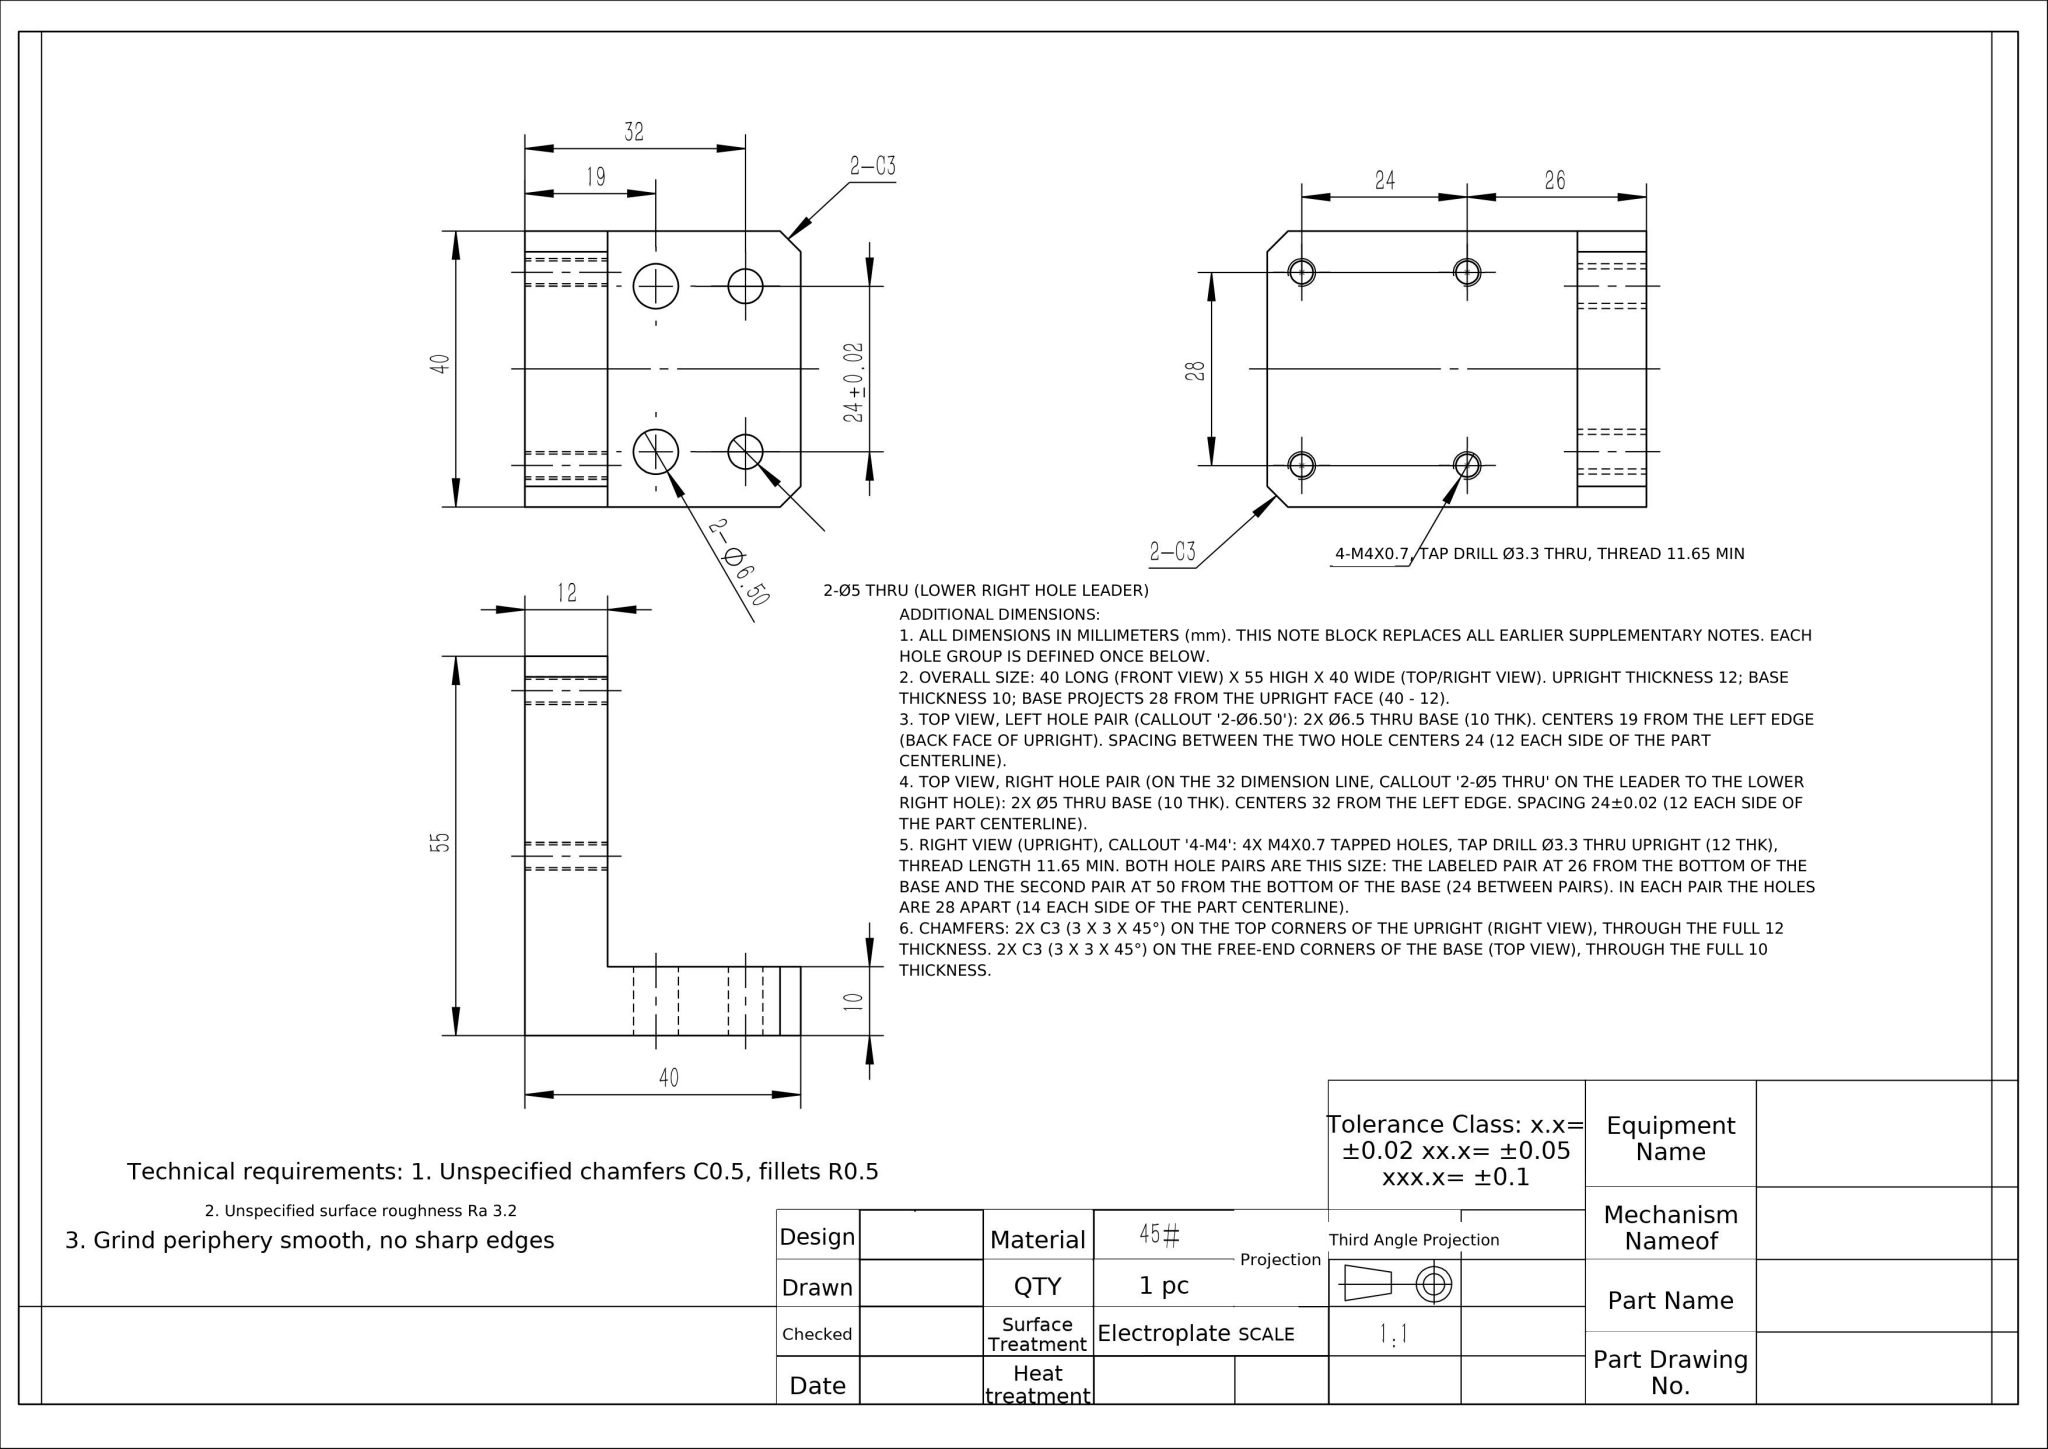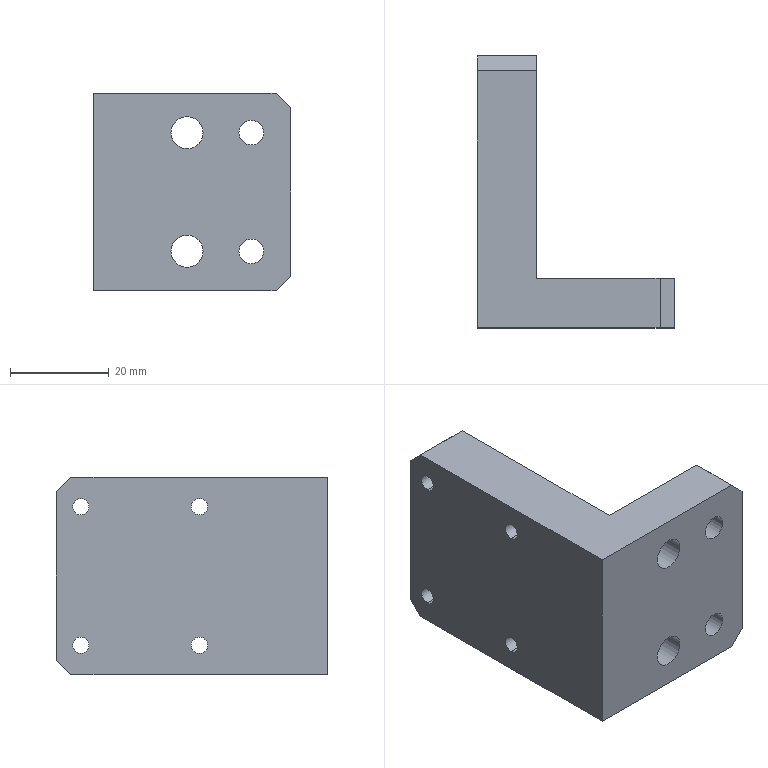Part | NX | mm | 1 solid | 28 faces | box 40 x 55 x 40 mm | volume 35935 mm3 | cylinder 16 | plane 12 | commonest cylinder face diameters 3.3 x8 6.5 x4 5 x4
STEP:
#1=CARTESIAN_POINT('',(12.,50.,-15.65));
#2=VERTEX_POINT('',#1);
#3=CARTESIAN_POINT('',(12.,50.,-12.35));
#4=VERTEX_POINT('',#3);
#5=CARTESIAN_POINT('',(12.,50.,-14.));
#6=DIRECTION('',(-1.,0.,0.));
#7=DIRECTION('',(0.,0.,1.));
#8=AXIS2_PLACEMENT_3D('',#5,#6,#7);
#9=CIRCLE('',#8,1.65);
#10=EDGE_CURVE('',#2,#4,#9,.T.);
#11=ORIENTED_EDGE('',*,*,#10,.F.);
#12=CARTESIAN_POINT('',(-0.,50.,-15.65));
#13=VERTEX_POINT('',#12);
#14=CARTESIAN_POINT('',(0.,50.,-15.65));
#15=DIRECTION('',(-1.,0.,0.));
#16=VECTOR('',#15,1000.);
#17=LINE('',#14,#16);
#18=EDGE_CURVE('',#2,#13,#17,.T.);
#19=ORIENTED_EDGE('',*,*,#18,.T.);
#20=CARTESIAN_POINT('',(-0.,50.,-12.35));
#21=VERTEX_POINT('',#20);
#22=CARTESIAN_POINT('',(-0.,50.,-14.));
#23=DIRECTION('',(-1.,0.,0.));
#24=DIRECTION('',(0.,0.,1.));
#25=AXIS2_PLACEMENT_3D('',#22,#23,#24);
#26=CIRCLE('',#25,1.65);
#27=EDGE_CURVE('',#13,#21,#26,.T.);
#28=ORIENTED_EDGE('',*,*,#27,.T.);
#29=CARTESIAN_POINT('',(0.,50.,-12.35));
#30=DIRECTION('',(-1.,0.,0.));
#31=VECTOR('',#30,1000.);
#32=LINE('',#29,#31);
#33=EDGE_CURVE('',#4,#21,#32,.T.);
#34=ORIENTED_EDGE('',*,*,#33,.F.);
#35=EDGE_LOOP('',(#11,#19,#28,#34));
#36=FACE_OUTER_BOUND('',#35,.T.);
#37=CARTESIAN_POINT('',(0.,50.,-14.));
#38=DIRECTION('',(-1.,0.,0.));
#39=DIRECTION('',(0.,0.,1.));
#40=AXIS2_PLACEMENT_3D('',#37,#38,#39);
#41=CYLINDRICAL_SURFACE('',#40,1.65);
#42=ADVANCED_FACE('',(#36),#41,.F.);
#43=CARTESIAN_POINT('',(12.,50.,12.35));
#44=VERTEX_POINT('',#43);
#45=CARTESIAN_POINT('',(12.,50.,15.65));
#46=VERTEX_POINT('',#45);
#47=CARTESIAN_POINT('',(12.,50.,14.));
#48=DIRECTION('',(-1.,0.,0.));
#49=DIRECTION('',(0.,0.,1.));
#50=AXIS2_PLACEMENT_3D('',#47,#48,#49);
#51=CIRCLE('',#50,1.65);
#52=EDGE_CURVE('',#44,#46,#51,.T.);
#53=ORIENTED_EDGE('',*,*,#52,.F.);
#54=CARTESIAN_POINT('',(-0.,50.,12.35));
#55=VERTEX_POINT('',#54);
#56=CARTESIAN_POINT('',(0.,50.,12.35));
#57=DIRECTION('',(-1.,0.,0.));
#58=VECTOR('',#57,1000.);
#59=LINE('',#56,#58);
#60=EDGE_CURVE('',#44,#55,#59,.T.);
#61=ORIENTED_EDGE('',*,*,#60,.T.);
#62=CARTESIAN_POINT('',(-0.,50.,15.65));
#63=VERTEX_POINT('',#62);
#64=CARTESIAN_POINT('',(-0.,50.,14.));
#65=DIRECTION('',(-1.,0.,0.));
#66=DIRECTION('',(0.,0.,1.));
#67=AXIS2_PLACEMENT_3D('',#64,#65,#66);
#68=CIRCLE('',#67,1.65);
#69=EDGE_CURVE('',#55,#63,#68,.T.);
#70=ORIENTED_EDGE('',*,*,#69,.T.);
#71=CARTESIAN_POINT('',(0.,50.,15.65));
#72=DIRECTION('',(-1.,0.,0.));
#73=VECTOR('',#72,1000.);
#74=LINE('',#71,#73);
#75=EDGE_CURVE('',#46,#63,#74,.T.);
#76=ORIENTED_EDGE('',*,*,#75,.F.);
#77=EDGE_LOOP('',(#53,#61,#70,#76));
#78=FACE_OUTER_BOUND('',#77,.T.);
#79=CARTESIAN_POINT('',(0.,50.,14.));
#80=DIRECTION('',(-1.,0.,0.));
#81=DIRECTION('',(0.,0.,1.));
#82=AXIS2_PLACEMENT_3D('',#79,#80,#81);
#83=CYLINDRICAL_SURFACE('',#82,1.65);
#84=ADVANCED_FACE('',(#78),#83,.F.);
#85=CARTESIAN_POINT('',(12.,26.,12.35));
#86=VERTEX_POINT('',#85);
#87=CARTESIAN_POINT('',(12.,26.,15.65));
#88=VERTEX_POINT('',#87);
#89=CARTESIAN_POINT('',(12.,26.,14.));
#90=DIRECTION('',(-1.,0.,0.));
#91=DIRECTION('',(0.,0.,1.));
#92=AXIS2_PLACEMENT_3D('',#89,#90,#91);
#93=CIRCLE('',#92,1.65);
#94=EDGE_CURVE('',#86,#88,#93,.T.);
#95=ORIENTED_EDGE('',*,*,#94,.F.);
#96=CARTESIAN_POINT('',(-0.,26.,12.35));
#97=VERTEX_POINT('',#96);
#98=CARTESIAN_POINT('',(0.,26.,12.35));
#99=DIRECTION('',(-1.,0.,0.));
#100=VECTOR('',#99,1000.);
#101=LINE('',#98,#100);
#102=EDGE_CURVE('',#86,#97,#101,.T.);
#103=ORIENTED_EDGE('',*,*,#102,.T.);
#104=CARTESIAN_POINT('',(-0.,26.,15.65));
#105=VERTEX_POINT('',#104);
#106=CARTESIAN_POINT('',(-0.,26.,14.));
#107=DIRECTION('',(-1.,0.,0.));
#108=DIRECTION('',(0.,0.,1.));
#109=AXIS2_PLACEMENT_3D('',#106,#107,#108);
#110=CIRCLE('',#109,1.65);
#111=EDGE_CURVE('',#97,#105,#110,.T.);
#112=ORIENTED_EDGE('',*,*,#111,.T.);
#113=CARTESIAN_POINT('',(0.,26.,15.65));
#114=DIRECTION('',(-1.,0.,0.));
#115=VECTOR('',#114,1000.);
#116=LINE('',#113,#115);
#117=EDGE_CURVE('',#88,#105,#116,.T.);
#118=ORIENTED_EDGE('',*,*,#117,.F.);
#119=EDGE_LOOP('',(#95,#103,#112,#118));
#120=FACE_OUTER_BOUND('',#119,.T.);
#121=CARTESIAN_POINT('',(0.,26.,14.));
#122=DIRECTION('',(-1.,0.,0.));
#123=DIRECTION('',(0.,0.,1.));
#124=AXIS2_PLACEMENT_3D('',#121,#122,#123);
#125=CYLINDRICAL_SURFACE('',#124,1.65);
#126=ADVANCED_FACE('',(#120),#125,.F.);
#127=CARTESIAN_POINT('',(12.,26.,-15.65));
#128=VERTEX_POINT('',#127);
#129=CARTESIAN_POINT('',(12.,26.,-12.35));
#130=VERTEX_POINT('',#129);
#131=CARTESIAN_POINT('',(12.,26.,-14.));
#132=DIRECTION('',(-1.,0.,0.));
#133=DIRECTION('',(0.,0.,1.));
#134=AXIS2_PLACEMENT_3D('',#131,#132,#133);
#135=CIRCLE('',#134,1.65);
#136=EDGE_CURVE('',#128,#130,#135,.T.);
#137=ORIENTED_EDGE('',*,*,#136,.F.);
#138=CARTESIAN_POINT('',(-0.,26.,-15.65));
#139=VERTEX_POINT('',#138);
#140=CARTESIAN_POINT('',(0.,26.,-15.65));
#141=DIRECTION('',(-1.,0.,0.));
#142=VECTOR('',#141,1000.);
#143=LINE('',#140,#142);
#144=EDGE_CURVE('',#128,#139,#143,.T.);
#145=ORIENTED_EDGE('',*,*,#144,.T.);
#146=CARTESIAN_POINT('',(-0.,26.,-12.35));
#147=VERTEX_POINT('',#146);
#148=CARTESIAN_POINT('',(-0.,26.,-14.));
#149=DIRECTION('',(-1.,0.,0.));
#150=DIRECTION('',(0.,0.,1.));
#151=AXIS2_PLACEMENT_3D('',#148,#149,#150);
#152=CIRCLE('',#151,1.65);
#153=EDGE_CURVE('',#139,#147,#152,.T.);
#154=ORIENTED_EDGE('',*,*,#153,.T.);
#155=CARTESIAN_POINT('',(0.,26.,-12.35));
#156=DIRECTION('',(-1.,0.,0.));
#157=VECTOR('',#156,1000.);
#158=LINE('',#155,#157);
#159=EDGE_CURVE('',#130,#147,#158,.T.);
#160=ORIENTED_EDGE('',*,*,#159,.F.);
#161=EDGE_LOOP('',(#137,#145,#154,#160));
#162=FACE_OUTER_BOUND('',#161,.T.);
#163=CARTESIAN_POINT('',(0.,26.,-14.));
#164=DIRECTION('',(-1.,0.,0.));
#165=DIRECTION('',(0.,0.,1.));
#166=AXIS2_PLACEMENT_3D('',#163,#164,#165);
#167=CYLINDRICAL_SURFACE('',#166,1.65);
#168=ADVANCED_FACE('',(#162),#167,.F.);
#169=CARTESIAN_POINT('',(22.25,-0.,12.));
#170=VERTEX_POINT('',#169);
#171=CARTESIAN_POINT('',(15.75,-0.,12.));
#172=VERTEX_POINT('',#171);
#173=CARTESIAN_POINT('',(19.,-0.,12.));
#174=DIRECTION('',(-0.,1.,0.));
#175=DIRECTION('',(1.,0.,0.));
#176=AXIS2_PLACEMENT_3D('',#173,#174,#175);
#177=CIRCLE('',#176,3.25);
#178=EDGE_CURVE('',#170,#172,#177,.T.);
#179=ORIENTED_EDGE('',*,*,#178,.F.);
#180=CARTESIAN_POINT('',(22.25,10.,12.));
#181=VERTEX_POINT('',#180);
#182=CARTESIAN_POINT('',(22.25,-0.,12.));
#183=DIRECTION('',(-0.,1.,0.));
#184=VECTOR('',#183,1000.);
#185=LINE('',#182,#184);
#186=EDGE_CURVE('',#170,#181,#185,.T.);
#187=ORIENTED_EDGE('',*,*,#186,.T.);
#188=CARTESIAN_POINT('',(15.75,10.,12.));
#189=VERTEX_POINT('',#188);
#190=CARTESIAN_POINT('',(19.,10.,12.));
#191=DIRECTION('',(-0.,1.,0.));
#192=DIRECTION('',(1.,0.,0.));
#193=AXIS2_PLACEMENT_3D('',#190,#191,#192);
#194=CIRCLE('',#193,3.25);
#195=EDGE_CURVE('',#181,#189,#194,.T.);
#196=ORIENTED_EDGE('',*,*,#195,.T.);
#197=CARTESIAN_POINT('',(15.75,-0.,12.));
#198=DIRECTION('',(-0.,1.,0.));
#199=VECTOR('',#198,1000.);
#200=LINE('',#197,#199);
#201=EDGE_CURVE('',#172,#189,#200,.T.);
#202=ORIENTED_EDGE('',*,*,#201,.F.);
#203=EDGE_LOOP('',(#179,#187,#196,#202));
#204=FACE_OUTER_BOUND('',#203,.T.);
#205=CARTESIAN_POINT('',(19.,-0.,12.));
#206=DIRECTION('',(-0.,1.,0.));
#207=DIRECTION('',(-1.,-0.,0.));
#208=AXIS2_PLACEMENT_3D('',#205,#206,#207);
#209=CYLINDRICAL_SURFACE('',#208,3.25);
#210=ADVANCED_FACE('',(#204),#209,.F.);
#211=CARTESIAN_POINT('',(34.5,-0.,12.));
#212=VERTEX_POINT('',#211);
#213=CARTESIAN_POINT('',(29.5,-0.,12.));
#214=VERTEX_POINT('',#213);
#215=CARTESIAN_POINT('',(32.,-0.,12.));
#216=DIRECTION('',(-0.,1.,0.));
#217=DIRECTION('',(1.,0.,0.));
#218=AXIS2_PLACEMENT_3D('',#215,#216,#217);
#219=CIRCLE('',#218,2.5);
#220=EDGE_CURVE('',#212,#214,#219,.T.);
#221=ORIENTED_EDGE('',*,*,#220,.F.);
#222=CARTESIAN_POINT('',(34.5,10.,12.));
#223=VERTEX_POINT('',#222);
#224=CARTESIAN_POINT('',(34.5,-0.,12.));
#225=DIRECTION('',(-0.,1.,0.));
#226=VECTOR('',#225,1000.);
#227=LINE('',#224,#226);
#228=EDGE_CURVE('',#212,#223,#227,.T.);
#229=ORIENTED_EDGE('',*,*,#228,.T.);
#230=CARTESIAN_POINT('',(29.5,10.,12.));
#231=VERTEX_POINT('',#230);
#232=CARTESIAN_POINT('',(32.,10.,12.));
#233=DIRECTION('',(-0.,1.,0.));
#234=DIRECTION('',(1.,0.,0.));
#235=AXIS2_PLACEMENT_3D('',#232,#233,#234);
#236=CIRCLE('',#235,2.5);
#237=EDGE_CURVE('',#223,#231,#236,.T.);
#238=ORIENTED_EDGE('',*,*,#237,.T.);
#239=CARTESIAN_POINT('',(29.5,-0.,12.));
#240=DIRECTION('',(-0.,1.,0.));
#241=VECTOR('',#240,1000.);
#242=LINE('',#239,#241);
#243=EDGE_CURVE('',#214,#231,#242,.T.);
#244=ORIENTED_EDGE('',*,*,#243,.F.);
#245=EDGE_LOOP('',(#221,#229,#238,#244));
#246=FACE_OUTER_BOUND('',#245,.T.);
#247=CARTESIAN_POINT('',(32.,-0.,12.));
#248=DIRECTION('',(-0.,1.,0.));
#249=DIRECTION('',(-1.,-0.,0.));
#250=AXIS2_PLACEMENT_3D('',#247,#248,#249);
#251=CYLINDRICAL_SURFACE('',#250,2.5);
#252=ADVANCED_FACE('',(#246),#251,.F.);
#253=CARTESIAN_POINT('',(34.5,-0.,-12.));
#254=VERTEX_POINT('',#253);
#255=CARTESIAN_POINT('',(29.5,-0.,-12.));
#256=VERTEX_POINT('',#255);
#257=CARTESIAN_POINT('',(32.,-0.,-12.));
#258=DIRECTION('',(-0.,1.,0.));
#259=DIRECTION('',(-1.,-0.,0.));
#260=AXIS2_PLACEMENT_3D('',#257,#258,#259);
#261=CIRCLE('',#260,2.5);
#262=EDGE_CURVE('',#254,#256,#261,.T.);
#263=ORIENTED_EDGE('',*,*,#262,.F.);
#264=CARTESIAN_POINT('',(34.5,10.,-12.));
#265=VERTEX_POINT('',#264);
#266=CARTESIAN_POINT('',(34.5,-0.,-12.));
#267=DIRECTION('',(-0.,1.,0.));
#268=VECTOR('',#267,1000.);
#269=LINE('',#266,#268);
#270=EDGE_CURVE('',#254,#265,#269,.T.);
#271=ORIENTED_EDGE('',*,*,#270,.T.);
#272=CARTESIAN_POINT('',(29.5,10.,-12.));
#273=VERTEX_POINT('',#272);
#274=CARTESIAN_POINT('',(32.,10.,-12.));
#275=DIRECTION('',(-0.,1.,0.));
#276=DIRECTION('',(-1.,0.,0.));
#277=AXIS2_PLACEMENT_3D('',#274,#275,#276);
#278=CIRCLE('',#277,2.5);
#279=EDGE_CURVE('',#265,#273,#278,.T.);
#280=ORIENTED_EDGE('',*,*,#279,.T.);
#281=CARTESIAN_POINT('',(29.5,-0.,-12.));
#282=DIRECTION('',(-0.,1.,0.));
#283=VECTOR('',#282,1000.);
#284=LINE('',#281,#283);
#285=EDGE_CURVE('',#256,#273,#284,.T.);
#286=ORIENTED_EDGE('',*,*,#285,.F.);
#287=EDGE_LOOP('',(#263,#271,#280,#286));
#288=FACE_OUTER_BOUND('',#287,.T.);
#289=CARTESIAN_POINT('',(32.,-0.,-12.));
#290=DIRECTION('',(-0.,1.,0.));
#291=DIRECTION('',(-1.,-0.,0.));
#292=AXIS2_PLACEMENT_3D('',#289,#290,#291);
#293=CYLINDRICAL_SURFACE('',#292,2.5);
#294=ADVANCED_FACE('',(#288),#293,.F.);
#295=CARTESIAN_POINT('',(22.25,-0.,-12.));
#296=VERTEX_POINT('',#295);
#297=CARTESIAN_POINT('',(15.75,-0.,-12.));
#298=VERTEX_POINT('',#297);
#299=CARTESIAN_POINT('',(19.,-0.,-12.));
#300=DIRECTION('',(-0.,1.,0.));
#301=DIRECTION('',(-1.,-0.,0.));
#302=AXIS2_PLACEMENT_3D('',#299,#300,#301);
#303=CIRCLE('',#302,3.25);
#304=EDGE_CURVE('',#296,#298,#303,.T.);
#305=ORIENTED_EDGE('',*,*,#304,.F.);
#306=CARTESIAN_POINT('',(22.25,10.,-12.));
#307=VERTEX_POINT('',#306);
#308=CARTESIAN_POINT('',(22.25,-0.,-12.));
#309=DIRECTION('',(-0.,1.,0.));
#310=VECTOR('',#309,1000.);
#311=LINE('',#308,#310);
#312=EDGE_CURVE('',#296,#307,#311,.T.);
#313=ORIENTED_EDGE('',*,*,#312,.T.);
#314=CARTESIAN_POINT('',(15.75,10.,-12.));
#315=VERTEX_POINT('',#314);
#316=CARTESIAN_POINT('',(19.,10.,-12.));
#317=DIRECTION('',(-0.,1.,0.));
#318=DIRECTION('',(-1.,0.,0.));
#319=AXIS2_PLACEMENT_3D('',#316,#317,#318);
#320=CIRCLE('',#319,3.25);
#321=EDGE_CURVE('',#307,#315,#320,.T.);
#322=ORIENTED_EDGE('',*,*,#321,.T.);
#323=CARTESIAN_POINT('',(15.75,-0.,-12.));
#324=DIRECTION('',(-0.,1.,0.));
#325=VECTOR('',#324,1000.);
#326=LINE('',#323,#325);
#327=EDGE_CURVE('',#298,#315,#326,.T.);
#328=ORIENTED_EDGE('',*,*,#327,.F.);
#329=EDGE_LOOP('',(#305,#313,#322,#328));
#330=FACE_OUTER_BOUND('',#329,.T.);
#331=CARTESIAN_POINT('',(19.,-0.,-12.));
#332=DIRECTION('',(-0.,1.,0.));
#333=DIRECTION('',(-1.,-0.,0.));
#334=AXIS2_PLACEMENT_3D('',#331,#332,#333);
#335=CYLINDRICAL_SURFACE('',#334,3.25);
#336=ADVANCED_FACE('',(#330),#335,.F.);
#337=CARTESIAN_POINT('',(12.,55.,17.));
#338=VERTEX_POINT('',#337);
#339=CARTESIAN_POINT('',(12.,55.,-17.));
#340=VERTEX_POINT('',#339);
#341=CARTESIAN_POINT('',(12.,55.,20.));
#342=DIRECTION('',(0.,0.,-1.));
#343=VECTOR('',#342,1000.);
#344=LINE('',#341,#343);
#345=EDGE_CURVE('',#338,#340,#344,.T.);
#346=ORIENTED_EDGE('',*,*,#345,.T.);
#347=CARTESIAN_POINT('',(0.,55.,-17.));
#348=VERTEX_POINT('',#347);
#349=CARTESIAN_POINT('',(12.,55.,-17.));
#350=DIRECTION('',(-1.,0.,0.));
#351=VECTOR('',#350,1000.);
#352=LINE('',#349,#351);
#353=EDGE_CURVE('',#340,#348,#352,.T.);
#354=ORIENTED_EDGE('',*,*,#353,.T.);
#355=CARTESIAN_POINT('',(0.,55.,17.));
#356=VERTEX_POINT('',#355);
#357=CARTESIAN_POINT('',(0.,55.,20.));
#358=DIRECTION('',(0.,0.,-1.));
#359=VECTOR('',#358,1000.);
#360=LINE('',#357,#359);
#361=EDGE_CURVE('',#356,#348,#360,.T.);
#362=ORIENTED_EDGE('',*,*,#361,.F.);
#363=CARTESIAN_POINT('',(12.,55.,17.));
#364=DIRECTION('',(1.,0.,0.));
#365=VECTOR('',#364,1000.);
#366=LINE('',#363,#365);
#367=EDGE_CURVE('',#356,#338,#366,.T.);
#368=ORIENTED_EDGE('',*,*,#367,.T.);
#369=EDGE_LOOP('',(#346,#354,#362,#368));
#370=FACE_OUTER_BOUND('',#369,.T.);
#371=CARTESIAN_POINT('',(12.,55.,20.));
#372=DIRECTION('',(0.,-1.,0.));
#373=DIRECTION('',(0.,0.,-1.));
#374=AXIS2_PLACEMENT_3D('',#371,#372,#373);
#375=PLANE('',#374);
#376=ADVANCED_FACE('',(#370),#375,.F.);
#377=CARTESIAN_POINT('',(-0.,50.,-14.));
#378=DIRECTION('',(-1.,0.,0.));
#379=DIRECTION('',(0.,0.,1.));
#380=AXIS2_PLACEMENT_3D('',#377,#378,#379);
#381=CIRCLE('',#380,1.65);
#382=EDGE_CURVE('',#21,#13,#381,.T.);
#383=ORIENTED_EDGE('',*,*,#382,.F.);
#384=ORIENTED_EDGE('',*,*,#27,.F.);
#385=EDGE_LOOP('',(#383,#384));
#386=FACE_BOUND('',#385,.T.);
#387=CARTESIAN_POINT('',(-0.,50.,14.));
#388=DIRECTION('',(-1.,0.,0.));
#389=DIRECTION('',(0.,0.,1.));
#390=AXIS2_PLACEMENT_3D('',#387,#388,#389);
#391=CIRCLE('',#390,1.65);
#392=EDGE_CURVE('',#63,#55,#391,.T.);
#393=ORIENTED_EDGE('',*,*,#392,.F.);
#394=ORIENTED_EDGE('',*,*,#69,.F.);
#395=EDGE_LOOP('',(#393,#394));
#396=FACE_BOUND('',#395,.T.);
#397=CARTESIAN_POINT('',(-0.,26.,14.));
#398=DIRECTION('',(-1.,0.,0.));
#399=DIRECTION('',(0.,0.,1.));
#400=AXIS2_PLACEMENT_3D('',#397,#398,#399);
#401=CIRCLE('',#400,1.65);
#402=EDGE_CURVE('',#105,#97,#401,.T.);
#403=ORIENTED_EDGE('',*,*,#402,.F.);
#404=ORIENTED_EDGE('',*,*,#111,.F.);
#405=EDGE_LOOP('',(#403,#404));
#406=FACE_BOUND('',#405,.T.);
#407=CARTESIAN_POINT('',(-0.,26.,-14.));
#408=DIRECTION('',(-1.,0.,0.));
#409=DIRECTION('',(0.,0.,1.));
#410=AXIS2_PLACEMENT_3D('',#407,#408,#409);
#411=CIRCLE('',#410,1.65);
#412=EDGE_CURVE('',#147,#139,#411,.T.);
#413=ORIENTED_EDGE('',*,*,#412,.F.);
#414=ORIENTED_EDGE('',*,*,#153,.F.);
#415=EDGE_LOOP('',(#413,#414));
#416=FACE_BOUND('',#415,.T.);
#417=ORIENTED_EDGE('',*,*,#361,.T.);
#418=CARTESIAN_POINT('',(0.,52.,-20.));
#419=VERTEX_POINT('',#418);
#420=CARTESIAN_POINT('',(0.,55.,-17.));
#421=DIRECTION('',(-0.,-0.7071,-0.7071));
#422=VECTOR('',#421,1000.);
#423=LINE('',#420,#422);
#424=EDGE_CURVE('',#348,#419,#423,.T.);
#425=ORIENTED_EDGE('',*,*,#424,.T.);
#426=CARTESIAN_POINT('',(0.,0.,-20.));
#427=VERTEX_POINT('',#426);
#428=CARTESIAN_POINT('',(0.,55.,-20.));
#429=DIRECTION('',(-0.,-1.,0.));
#430=VECTOR('',#429,1000.);
#431=LINE('',#428,#430);
#432=EDGE_CURVE('',#419,#427,#431,.T.);
#433=ORIENTED_EDGE('',*,*,#432,.T.);
#434=CARTESIAN_POINT('',(0.,0.,20.));
#435=VERTEX_POINT('',#434);
#436=CARTESIAN_POINT('',(0.,0.,20.));
#437=DIRECTION('',(0.,0.,-1.));
#438=VECTOR('',#437,1000.);
#439=LINE('',#436,#438);
#440=EDGE_CURVE('',#435,#427,#439,.T.);
#441=ORIENTED_EDGE('',*,*,#440,.F.);
#442=CARTESIAN_POINT('',(0.,52.,20.));
#443=VERTEX_POINT('',#442);
#444=CARTESIAN_POINT('',(0.,55.,20.));
#445=DIRECTION('',(-0.,-1.,0.));
#446=VECTOR('',#445,1000.);
#447=LINE('',#444,#446);
#448=EDGE_CURVE('',#443,#435,#447,.T.);
#449=ORIENTED_EDGE('',*,*,#448,.F.);
#450=CARTESIAN_POINT('',(0.,52.,20.));
#451=DIRECTION('',(0.,0.7071,-0.7071));
#452=VECTOR('',#451,1000.);
#453=LINE('',#450,#452);
#454=EDGE_CURVE('',#443,#356,#453,.T.);
#455=ORIENTED_EDGE('',*,*,#454,.T.);
#456=EDGE_LOOP('',(#417,#425,#433,#441,#449,#455));
#457=FACE_OUTER_BOUND('',#456,.T.);
#458=CARTESIAN_POINT('',(0.,55.,20.));
#459=DIRECTION('',(1.,-0.,0.));
#460=DIRECTION('',(0.,1.,0.));
#461=AXIS2_PLACEMENT_3D('',#458,#459,#460);
#462=PLANE('',#461);
#463=ADVANCED_FACE('',(#386,#396,#406,#416,#457),#462,.F.);
#464=CARTESIAN_POINT('',(19.,-0.,12.));
#465=DIRECTION('',(-0.,1.,0.));
#466=DIRECTION('',(1.,0.,0.));
#467=AXIS2_PLACEMENT_3D('',#464,#465,#466);
#468=CIRCLE('',#467,3.25);
#469=EDGE_CURVE('',#172,#170,#468,.T.);
#470=ORIENTED_EDGE('',*,*,#469,.T.);
#471=ORIENTED_EDGE('',*,*,#178,.T.);
#472=EDGE_LOOP('',(#470,#471));
#473=FACE_BOUND('',#472,.T.);
#474=CARTESIAN_POINT('',(32.,-0.,12.));
#475=DIRECTION('',(-0.,1.,0.));
#476=DIRECTION('',(1.,0.,0.));
#477=AXIS2_PLACEMENT_3D('',#474,#475,#476);
#478=CIRCLE('',#477,2.5);
#479=EDGE_CURVE('',#214,#212,#478,.T.);
#480=ORIENTED_EDGE('',*,*,#479,.T.);
#481=ORIENTED_EDGE('',*,*,#220,.T.);
#482=EDGE_LOOP('',(#480,#481));
#483=FACE_BOUND('',#482,.T.);
#484=CARTESIAN_POINT('',(32.,-0.,-12.));
#485=DIRECTION('',(-0.,1.,0.));
#486=DIRECTION('',(-1.,-0.,0.));
#487=AXIS2_PLACEMENT_3D('',#484,#485,#486);
#488=CIRCLE('',#487,2.5);
#489=EDGE_CURVE('',#256,#254,#488,.T.);
#490=ORIENTED_EDGE('',*,*,#489,.T.);
#491=ORIENTED_EDGE('',*,*,#262,.T.);
#492=EDGE_LOOP('',(#490,#491));
#493=FACE_BOUND('',#492,.T.);
#494=CARTESIAN_POINT('',(19.,-0.,-12.));
#495=DIRECTION('',(-0.,1.,0.));
#496=DIRECTION('',(-1.,-0.,0.));
#497=AXIS2_PLACEMENT_3D('',#494,#495,#496);
#498=CIRCLE('',#497,3.25);
#499=EDGE_CURVE('',#298,#296,#498,.T.);
#500=ORIENTED_EDGE('',*,*,#499,.T.);
#501=ORIENTED_EDGE('',*,*,#304,.T.);
#502=EDGE_LOOP('',(#500,#501));
#503=FACE_BOUND('',#502,.T.);
#504=CARTESIAN_POINT('',(37.,0.,-20.));
#505=VERTEX_POINT('',#504);
#506=CARTESIAN_POINT('',(0.,0.,-20.));
#507=DIRECTION('',(1.,0.,0.));
#508=VECTOR('',#507,1000.);
#509=LINE('',#506,#508);
#510=EDGE_CURVE('',#427,#505,#509,.T.);
#511=ORIENTED_EDGE('',*,*,#510,.T.);
#512=CARTESIAN_POINT('',(40.,0.,-17.));
#513=VERTEX_POINT('',#512);
#514=CARTESIAN_POINT('',(40.,0.,-17.));
#515=DIRECTION('',(0.7071,0.,0.7071));
#516=VECTOR('',#515,1000.);
#517=LINE('',#514,#516);
#518=EDGE_CURVE('',#505,#513,#517,.T.);
#519=ORIENTED_EDGE('',*,*,#518,.T.);
#520=CARTESIAN_POINT('',(40.,0.,17.));
#521=VERTEX_POINT('',#520);
#522=CARTESIAN_POINT('',(40.,0.,20.));
#523=DIRECTION('',(0.,0.,-1.));
#524=VECTOR('',#523,1000.);
#525=LINE('',#522,#524);
#526=EDGE_CURVE('',#521,#513,#525,.T.);
#527=ORIENTED_EDGE('',*,*,#526,.F.);
#528=CARTESIAN_POINT('',(37.,0.,20.));
#529=VERTEX_POINT('',#528);
#530=CARTESIAN_POINT('',(37.,0.,20.));
#531=DIRECTION('',(-0.7071,0.,0.7071));
#532=VECTOR('',#531,1000.);
#533=LINE('',#530,#532);
#534=EDGE_CURVE('',#521,#529,#533,.T.);
#535=ORIENTED_EDGE('',*,*,#534,.T.);
#536=CARTESIAN_POINT('',(0.,0.,20.));
#537=DIRECTION('',(1.,0.,0.));
#538=VECTOR('',#537,1000.);
#539=LINE('',#536,#538);
#540=EDGE_CURVE('',#435,#529,#539,.T.);
#541=ORIENTED_EDGE('',*,*,#540,.F.);
#542=ORIENTED_EDGE('',*,*,#440,.T.);
#543=EDGE_LOOP('',(#511,#519,#527,#535,#541,#542));
#544=FACE_OUTER_BOUND('',#543,.T.);
#545=CARTESIAN_POINT('',(0.,0.,20.));
#546=DIRECTION('',(0.,1.,0.));
#547=DIRECTION('',(0.,0.,1.));
#548=AXIS2_PLACEMENT_3D('',#545,#546,#547);
#549=PLANE('',#548);
#550=ADVANCED_FACE('',(#473,#483,#493,#503,#544),#549,.F.);
#551=ORIENTED_EDGE('',*,*,#526,.T.);
#552=CARTESIAN_POINT('',(40.,10.,-17.));
#553=VERTEX_POINT('',#552);
#554=CARTESIAN_POINT('',(40.,0.,-17.));
#555=DIRECTION('',(0.,1.,0.));
#556=VECTOR('',#555,1000.);
#557=LINE('',#554,#556);
#558=EDGE_CURVE('',#513,#553,#557,.T.);
#559=ORIENTED_EDGE('',*,*,#558,.T.);
#560=CARTESIAN_POINT('',(40.,10.,17.));
#561=VERTEX_POINT('',#560);
#562=CARTESIAN_POINT('',(40.,10.,20.));
#563=DIRECTION('',(0.,0.,-1.));
#564=VECTOR('',#563,1000.);
#565=LINE('',#562,#564);
#566=EDGE_CURVE('',#561,#553,#565,.T.);
#567=ORIENTED_EDGE('',*,*,#566,.F.);
#568=CARTESIAN_POINT('',(40.,0.,17.));
#569=DIRECTION('',(0.,-1.,0.));
#570=VECTOR('',#569,1000.);
#571=LINE('',#568,#570);
#572=EDGE_CURVE('',#561,#521,#571,.T.);
#573=ORIENTED_EDGE('',*,*,#572,.T.);
#574=EDGE_LOOP('',(#551,#559,#567,#573));
#575=FACE_OUTER_BOUND('',#574,.T.);
#576=CARTESIAN_POINT('',(40.,0.,20.));
#577=DIRECTION('',(-1.,0.,0.));
#578=DIRECTION('',(0.,0.,1.));
#579=AXIS2_PLACEMENT_3D('',#576,#577,#578);
#580=PLANE('',#579);
#581=ADVANCED_FACE('',(#575),#580,.F.);
#582=CARTESIAN_POINT('',(19.,10.,12.));
#583=DIRECTION('',(-0.,1.,0.));
#584=DIRECTION('',(1.,0.,0.));
#585=AXIS2_PLACEMENT_3D('',#582,#583,#584);
#586=CIRCLE('',#585,3.25);
#587=EDGE_CURVE('',#189,#181,#586,.T.);
#588=ORIENTED_EDGE('',*,*,#587,.F.);
#589=ORIENTED_EDGE('',*,*,#195,.F.);
#590=EDGE_LOOP('',(#588,#589));
#591=FACE_BOUND('',#590,.T.);
#592=CARTESIAN_POINT('',(32.,10.,12.));
#593=DIRECTION('',(-0.,1.,0.));
#594=DIRECTION('',(1.,0.,0.));
#595=AXIS2_PLACEMENT_3D('',#592,#593,#594);
#596=CIRCLE('',#595,2.5);
#597=EDGE_CURVE('',#231,#223,#596,.T.);
#598=ORIENTED_EDGE('',*,*,#597,.F.);
#599=ORIENTED_EDGE('',*,*,#237,.F.);
#600=EDGE_LOOP('',(#598,#599));
#601=FACE_BOUND('',#600,.T.);
#602=CARTESIAN_POINT('',(32.,10.,-12.));
#603=DIRECTION('',(-0.,1.,0.));
#604=DIRECTION('',(-1.,0.,0.));
#605=AXIS2_PLACEMENT_3D('',#602,#603,#604);
#606=CIRCLE('',#605,2.5);
#607=EDGE_CURVE('',#273,#265,#606,.T.);
#608=ORIENTED_EDGE('',*,*,#607,.F.);
#609=ORIENTED_EDGE('',*,*,#279,.F.);
#610=EDGE_LOOP('',(#608,#609));
#611=FACE_BOUND('',#610,.T.);
#612=CARTESIAN_POINT('',(19.,10.,-12.));
#613=DIRECTION('',(-0.,1.,0.));
#614=DIRECTION('',(-1.,0.,0.));
#615=AXIS2_PLACEMENT_3D('',#612,#613,#614);
#616=CIRCLE('',#615,3.25);
#617=EDGE_CURVE('',#315,#307,#616,.T.);
#618=ORIENTED_EDGE('',*,*,#617,.F.);
#619=ORIENTED_EDGE('',*,*,#321,.F.);
#620=EDGE_LOOP('',(#618,#619));
#621=FACE_BOUND('',#620,.T.);
#622=ORIENTED_EDGE('',*,*,#566,.T.);
#623=CARTESIAN_POINT('',(37.,10.,-20.));
#624=VERTEX_POINT('',#623);
#625=CARTESIAN_POINT('',(40.,10.,-17.));
#626=DIRECTION('',(-0.7071,-0.,-0.7071));
#627=VECTOR('',#626,1000.);
#628=LINE('',#625,#627);
#629=EDGE_CURVE('',#553,#624,#628,.T.);
#630=ORIENTED_EDGE('',*,*,#629,.T.);
#631=CARTESIAN_POINT('',(12.,10.,-20.));
#632=VERTEX_POINT('',#631);
#633=CARTESIAN_POINT('',(40.,10.,-20.));
#634=DIRECTION('',(-1.,-0.,0.));
#635=VECTOR('',#634,1000.);
#636=LINE('',#633,#635);
#637=EDGE_CURVE('',#624,#632,#636,.T.);
#638=ORIENTED_EDGE('',*,*,#637,.T.);
#639=CARTESIAN_POINT('',(12.,10.,20.));
#640=VERTEX_POINT('',#639);
#641=CARTESIAN_POINT('',(12.,10.,20.));
#642=DIRECTION('',(0.,0.,-1.));
#643=VECTOR('',#642,1000.);
#644=LINE('',#641,#643);
#645=EDGE_CURVE('',#640,#632,#644,.T.);
#646=ORIENTED_EDGE('',*,*,#645,.F.);
#647=CARTESIAN_POINT('',(37.,10.,20.));
#648=VERTEX_POINT('',#647);
#649=CARTESIAN_POINT('',(40.,10.,20.));
#650=DIRECTION('',(-1.,-0.,0.));
#651=VECTOR('',#650,1000.);
#652=LINE('',#649,#651);
#653=EDGE_CURVE('',#648,#640,#652,.T.);
#654=ORIENTED_EDGE('',*,*,#653,.F.);
#655=CARTESIAN_POINT('',(37.,10.,20.));
#656=DIRECTION('',(0.7071,0.,-0.7071));
#657=VECTOR('',#656,1000.);
#658=LINE('',#655,#657);
#659=EDGE_CURVE('',#648,#561,#658,.T.);
#660=ORIENTED_EDGE('',*,*,#659,.T.);
#661=EDGE_LOOP('',(#622,#630,#638,#646,#654,#660));
#662=FACE_OUTER_BOUND('',#661,.T.);
#663=CARTESIAN_POINT('',(40.,10.,20.));
#664=DIRECTION('',(0.,-1.,0.));
#665=DIRECTION('',(1.,0.,0.));
#666=AXIS2_PLACEMENT_3D('',#663,#664,#665);
#667=PLANE('',#666);
#668=ADVANCED_FACE('',(#591,#601,#611,#621,#662),#667,.F.);
#669=CARTESIAN_POINT('',(12.,50.,-14.));
#670=DIRECTION('',(-1.,0.,0.));
#671=DIRECTION('',(0.,0.,1.));
#672=AXIS2_PLACEMENT_3D('',#669,#670,#671);
#673=CIRCLE('',#672,1.65);
#674=EDGE_CURVE('',#4,#2,#673,.T.);
#675=ORIENTED_EDGE('',*,*,#674,.T.);
#676=ORIENTED_EDGE('',*,*,#10,.T.);
#677=EDGE_LOOP('',(#675,#676));
#678=FACE_BOUND('',#677,.T.);
#679=CARTESIAN_POINT('',(12.,50.,14.));
#680=DIRECTION('',(-1.,0.,0.));
#681=DIRECTION('',(0.,0.,1.));
#682=AXIS2_PLACEMENT_3D('',#679,#680,#681);
#683=CIRCLE('',#682,1.65);
#684=EDGE_CURVE('',#46,#44,#683,.T.);
#685=ORIENTED_EDGE('',*,*,#684,.T.);
#686=ORIENTED_EDGE('',*,*,#52,.T.);
#687=EDGE_LOOP('',(#685,#686));
#688=FACE_BOUND('',#687,.T.);
#689=CARTESIAN_POINT('',(12.,26.,14.));
#690=DIRECTION('',(-1.,0.,0.));
#691=DIRECTION('',(0.,0.,1.));
#692=AXIS2_PLACEMENT_3D('',#689,#690,#691);
#693=CIRCLE('',#692,1.65);
#694=EDGE_CURVE('',#88,#86,#693,.T.);
#695=ORIENTED_EDGE('',*,*,#694,.T.);
#696=ORIENTED_EDGE('',*,*,#94,.T.);
#697=EDGE_LOOP('',(#695,#696));
#698=FACE_BOUND('',#697,.T.);
#699=CARTESIAN_POINT('',(12.,26.,-14.));
#700=DIRECTION('',(-1.,0.,0.));
#701=DIRECTION('',(0.,0.,1.));
#702=AXIS2_PLACEMENT_3D('',#699,#700,#701);
#703=CIRCLE('',#702,1.65);
#704=EDGE_CURVE('',#130,#128,#703,.T.);
#705=ORIENTED_EDGE('',*,*,#704,.T.);
#706=ORIENTED_EDGE('',*,*,#136,.T.);
#707=EDGE_LOOP('',(#705,#706));
#708=FACE_BOUND('',#707,.T.);
#709=CARTESIAN_POINT('',(12.,52.,-20.));
#710=VERTEX_POINT('',#709);
#711=CARTESIAN_POINT('',(12.,10.,-20.));
#712=DIRECTION('',(0.,1.,0.));
#713=VECTOR('',#712,1000.);
#714=LINE('',#711,#713);
#715=EDGE_CURVE('',#632,#710,#714,.T.);
#716=ORIENTED_EDGE('',*,*,#715,.T.);
#717=CARTESIAN_POINT('',(12.,55.,-17.));
#718=DIRECTION('',(0.,0.7071,0.7071));
#719=VECTOR('',#718,1000.);
#720=LINE('',#717,#719);
#721=EDGE_CURVE('',#710,#340,#720,.T.);
#722=ORIENTED_EDGE('',*,*,#721,.T.);
#723=ORIENTED_EDGE('',*,*,#345,.F.);
#724=CARTESIAN_POINT('',(12.,52.,20.));
#725=VERTEX_POINT('',#724);
#726=CARTESIAN_POINT('',(12.,52.,20.));
#727=DIRECTION('',(0.,-0.7071,0.7071));
#728=VECTOR('',#727,1000.);
#729=LINE('',#726,#728);
#730=EDGE_CURVE('',#338,#725,#729,.T.);
#731=ORIENTED_EDGE('',*,*,#730,.T.);
#732=CARTESIAN_POINT('',(12.,10.,20.));
#733=DIRECTION('',(0.,1.,0.));
#734=VECTOR('',#733,1000.);
#735=LINE('',#732,#734);
#736=EDGE_CURVE('',#640,#725,#735,.T.);
#737=ORIENTED_EDGE('',*,*,#736,.F.);
#738=ORIENTED_EDGE('',*,*,#645,.T.);
#739=EDGE_LOOP('',(#716,#722,#723,#731,#737,#738));
#740=FACE_OUTER_BOUND('',#739,.T.);
#741=CARTESIAN_POINT('',(12.,10.,20.));
#742=DIRECTION('',(-1.,0.,0.));
#743=DIRECTION('',(0.,0.,1.));
#744=AXIS2_PLACEMENT_3D('',#741,#742,#743);
#745=PLANE('',#744);
#746=ADVANCED_FACE('',(#678,#688,#698,#708,#740),#745,.F.);
#747=ORIENTED_EDGE('',*,*,#736,.T.);
#748=CARTESIAN_POINT('',(0.,52.,20.));
#749=DIRECTION('',(-1.,0.,0.));
#750=VECTOR('',#749,1000.);
#751=LINE('',#748,#750);
#752=EDGE_CURVE('',#725,#443,#751,.T.);
#753=ORIENTED_EDGE('',*,*,#752,.T.);
#754=ORIENTED_EDGE('',*,*,#448,.T.);
#755=ORIENTED_EDGE('',*,*,#540,.T.);
#756=CARTESIAN_POINT('',(37.,10.,20.));
#757=DIRECTION('',(0.,1.,0.));
#758=VECTOR('',#757,1000.);
#759=LINE('',#756,#758);
#760=EDGE_CURVE('',#529,#648,#759,.T.);
#761=ORIENTED_EDGE('',*,*,#760,.T.);
#762=ORIENTED_EDGE('',*,*,#653,.T.);
#763=EDGE_LOOP('',(#747,#753,#754,#755,#761,#762));
#764=FACE_OUTER_BOUND('',#763,.T.);
#765=CARTESIAN_POINT('',(0.,0.,20.));
#766=DIRECTION('',(0.,0.,1.));
#767=DIRECTION('',(1.,0.,0.));
#768=AXIS2_PLACEMENT_3D('',#765,#766,#767);
#769=PLANE('',#768);
#770=ADVANCED_FACE('',(#764),#769,.T.);
#771=ORIENTED_EDGE('',*,*,#432,.F.);
#772=CARTESIAN_POINT('',(0.,52.,-20.));
#773=DIRECTION('',(1.,0.,0.));
#774=VECTOR('',#773,1000.);
#775=LINE('',#772,#774);
#776=EDGE_CURVE('',#419,#710,#775,.T.);
#777=ORIENTED_EDGE('',*,*,#776,.T.);
#778=ORIENTED_EDGE('',*,*,#715,.F.);
#779=ORIENTED_EDGE('',*,*,#637,.F.);
#780=CARTESIAN_POINT('',(37.,0.,-20.));
#781=DIRECTION('',(0.,-1.,0.));
#782=VECTOR('',#781,1000.);
#783=LINE('',#780,#782);
#784=EDGE_CURVE('',#624,#505,#783,.T.);
#785=ORIENTED_EDGE('',*,*,#784,.T.);
#786=ORIENTED_EDGE('',*,*,#510,.F.);
#787=EDGE_LOOP('',(#771,#777,#778,#779,#785,#786));
#788=FACE_OUTER_BOUND('',#787,.T.);
#789=CARTESIAN_POINT('',(0.,0.,-20.));
#790=DIRECTION('',(0.,0.,1.));
#791=DIRECTION('',(1.,0.,0.));
#792=AXIS2_PLACEMENT_3D('',#789,#790,#791);
#793=PLANE('',#792);
#794=ADVANCED_FACE('',(#788),#793,.F.);
#795=ORIENTED_EDGE('',*,*,#312,.F.);
#796=ORIENTED_EDGE('',*,*,#499,.F.);
#797=ORIENTED_EDGE('',*,*,#327,.T.);
#798=ORIENTED_EDGE('',*,*,#617,.T.);
#799=EDGE_LOOP('',(#795,#796,#797,#798));
#800=FACE_OUTER_BOUND('',#799,.T.);
#801=CARTESIAN_POINT('',(19.,-0.,-12.));
#802=DIRECTION('',(-0.,1.,0.));
#803=DIRECTION('',(-1.,-0.,0.));
#804=AXIS2_PLACEMENT_3D('',#801,#802,#803);
#805=CYLINDRICAL_SURFACE('',#804,3.25);
#806=ADVANCED_FACE('',(#800),#805,.F.);
#807=ORIENTED_EDGE('',*,*,#270,.F.);
#808=ORIENTED_EDGE('',*,*,#489,.F.);
#809=ORIENTED_EDGE('',*,*,#285,.T.);
#810=ORIENTED_EDGE('',*,*,#607,.T.);
#811=EDGE_LOOP('',(#807,#808,#809,#810));
#812=FACE_OUTER_BOUND('',#811,.T.);
#813=CARTESIAN_POINT('',(32.,-0.,-12.));
#814=DIRECTION('',(-0.,1.,0.));
#815=DIRECTION('',(-1.,-0.,0.));
#816=AXIS2_PLACEMENT_3D('',#813,#814,#815);
#817=CYLINDRICAL_SURFACE('',#816,2.5);
#818=ADVANCED_FACE('',(#812),#817,.F.);
#819=ORIENTED_EDGE('',*,*,#228,.F.);
#820=ORIENTED_EDGE('',*,*,#479,.F.);
#821=ORIENTED_EDGE('',*,*,#243,.T.);
#822=ORIENTED_EDGE('',*,*,#597,.T.);
#823=EDGE_LOOP('',(#819,#820,#821,#822));
#824=FACE_OUTER_BOUND('',#823,.T.);
#825=CARTESIAN_POINT('',(32.,-0.,12.));
#826=DIRECTION('',(-0.,1.,0.));
#827=DIRECTION('',(-1.,-0.,0.));
#828=AXIS2_PLACEMENT_3D('',#825,#826,#827);
#829=CYLINDRICAL_SURFACE('',#828,2.5);
#830=ADVANCED_FACE('',(#824),#829,.F.);
#831=ORIENTED_EDGE('',*,*,#186,.F.);
#832=ORIENTED_EDGE('',*,*,#469,.F.);
#833=ORIENTED_EDGE('',*,*,#201,.T.);
#834=ORIENTED_EDGE('',*,*,#587,.T.);
#835=EDGE_LOOP('',(#831,#832,#833,#834));
#836=FACE_OUTER_BOUND('',#835,.T.);
#837=CARTESIAN_POINT('',(19.,-0.,12.));
#838=DIRECTION('',(-0.,1.,0.));
#839=DIRECTION('',(-1.,-0.,0.));
#840=AXIS2_PLACEMENT_3D('',#837,#838,#839);
#841=CYLINDRICAL_SURFACE('',#840,3.25);
#842=ADVANCED_FACE('',(#836),#841,.F.);
#843=ORIENTED_EDGE('',*,*,#518,.F.);
#844=ORIENTED_EDGE('',*,*,#784,.F.);
#845=ORIENTED_EDGE('',*,*,#629,.F.);
#846=ORIENTED_EDGE('',*,*,#558,.F.);
#847=EDGE_LOOP('',(#843,#844,#845,#846));
#848=FACE_OUTER_BOUND('',#847,.T.);
#849=CARTESIAN_POINT('',(40.,0.,-17.));
#850=DIRECTION('',(-0.7071,0.,0.7071));
#851=DIRECTION('',(0.,1.,0.));
#852=AXIS2_PLACEMENT_3D('',#849,#850,#851);
#853=PLANE('',#852);
#854=ADVANCED_FACE('',(#848),#853,.F.);
#855=ORIENTED_EDGE('',*,*,#534,.F.);
#856=ORIENTED_EDGE('',*,*,#572,.F.);
#857=ORIENTED_EDGE('',*,*,#659,.F.);
#858=ORIENTED_EDGE('',*,*,#760,.F.);
#859=EDGE_LOOP('',(#855,#856,#857,#858));
#860=FACE_OUTER_BOUND('',#859,.T.);
#861=CARTESIAN_POINT('',(37.,0.,20.));
#862=DIRECTION('',(0.7071,0.,0.7071));
#863=DIRECTION('',(0.,-1.,0.));
#864=AXIS2_PLACEMENT_3D('',#861,#862,#863);
#865=PLANE('',#864);
#866=ADVANCED_FACE('',(#860),#865,.T.);
#867=ORIENTED_EDGE('',*,*,#721,.F.);
#868=ORIENTED_EDGE('',*,*,#776,.F.);
#869=ORIENTED_EDGE('',*,*,#424,.F.);
#870=ORIENTED_EDGE('',*,*,#353,.F.);
#871=EDGE_LOOP('',(#867,#868,#869,#870));
#872=FACE_OUTER_BOUND('',#871,.T.);
#873=CARTESIAN_POINT('',(12.,55.,-17.));
#874=DIRECTION('',(0.,-0.7071,0.7071));
#875=DIRECTION('',(-1.,0.,0.));
#876=AXIS2_PLACEMENT_3D('',#873,#874,#875);
#877=PLANE('',#876);
#878=ADVANCED_FACE('',(#872),#877,.F.);
#879=ORIENTED_EDGE('',*,*,#730,.F.);
#880=ORIENTED_EDGE('',*,*,#367,.F.);
#881=ORIENTED_EDGE('',*,*,#454,.F.);
#882=ORIENTED_EDGE('',*,*,#752,.F.);
#883=EDGE_LOOP('',(#879,#880,#881,#882));
#884=FACE_OUTER_BOUND('',#883,.T.);
#885=CARTESIAN_POINT('',(0.,52.,20.));
#886=DIRECTION('',(0.,0.7071,0.7071));
#887=DIRECTION('',(1.,0.,0.));
#888=AXIS2_PLACEMENT_3D('',#885,#886,#887);
#889=PLANE('',#888);
#890=ADVANCED_FACE('',(#884),#889,.T.);
#891=ORIENTED_EDGE('',*,*,#144,.F.);
#892=ORIENTED_EDGE('',*,*,#704,.F.);
#893=ORIENTED_EDGE('',*,*,#159,.T.);
#894=ORIENTED_EDGE('',*,*,#412,.T.);
#895=EDGE_LOOP('',(#891,#892,#893,#894));
#896=FACE_OUTER_BOUND('',#895,.T.);
#897=CARTESIAN_POINT('',(0.,26.,-14.));
#898=DIRECTION('',(-1.,0.,0.));
#899=DIRECTION('',(0.,0.,1.));
#900=AXIS2_PLACEMENT_3D('',#897,#898,#899);
#901=CYLINDRICAL_SURFACE('',#900,1.65);
#902=ADVANCED_FACE('',(#896),#901,.F.);
#903=ORIENTED_EDGE('',*,*,#102,.F.);
#904=ORIENTED_EDGE('',*,*,#694,.F.);
#905=ORIENTED_EDGE('',*,*,#117,.T.);
#906=ORIENTED_EDGE('',*,*,#402,.T.);
#907=EDGE_LOOP('',(#903,#904,#905,#906));
#908=FACE_OUTER_BOUND('',#907,.T.);
#909=CARTESIAN_POINT('',(0.,26.,14.));
#910=DIRECTION('',(-1.,0.,0.));
#911=DIRECTION('',(0.,0.,1.));
#912=AXIS2_PLACEMENT_3D('',#909,#910,#911);
#913=CYLINDRICAL_SURFACE('',#912,1.65);
#914=ADVANCED_FACE('',(#908),#913,.F.);
#915=ORIENTED_EDGE('',*,*,#60,.F.);
#916=ORIENTED_EDGE('',*,*,#684,.F.);
#917=ORIENTED_EDGE('',*,*,#75,.T.);
#918=ORIENTED_EDGE('',*,*,#392,.T.);
#919=EDGE_LOOP('',(#915,#916,#917,#918));
#920=FACE_OUTER_BOUND('',#919,.T.);
#921=CARTESIAN_POINT('',(0.,50.,14.));
#922=DIRECTION('',(-1.,0.,0.));
#923=DIRECTION('',(0.,0.,1.));
#924=AXIS2_PLACEMENT_3D('',#921,#922,#923);
#925=CYLINDRICAL_SURFACE('',#924,1.65);
#926=ADVANCED_FACE('',(#920),#925,.F.);
#927=ORIENTED_EDGE('',*,*,#18,.F.);
#928=ORIENTED_EDGE('',*,*,#674,.F.);
#929=ORIENTED_EDGE('',*,*,#33,.T.);
#930=ORIENTED_EDGE('',*,*,#382,.T.);
#931=EDGE_LOOP('',(#927,#928,#929,#930));
#932=FACE_OUTER_BOUND('',#931,.T.);
#933=CARTESIAN_POINT('',(0.,50.,-14.));
#934=DIRECTION('',(-1.,0.,0.));
#935=DIRECTION('',(0.,0.,1.));
#936=AXIS2_PLACEMENT_3D('',#933,#934,#935);
#937=CYLINDRICAL_SURFACE('',#936,1.65);
#938=ADVANCED_FACE('',(#932),#937,.F.);
#939=CLOSED_SHELL('',(#42,#84,#126,#168,#210,#252,#294,#336,#376,#463,#550,#581,#668,#746,#770,#794,#806,#818,#830,#842,#854,#866,#878,#890,#902,#914,#926,#938));
#940=MANIFOLD_SOLID_BREP('',#939);
#941=CARTESIAN_POINT('',(0.,0.,0.));
#942=DIRECTION('',(0.,0.,1.));
#943=DIRECTION('',(1.,0.,0.));
#944=AXIS2_PLACEMENT_3D('',#941,#942,#943);
#945=(LENGTH_UNIT()NAMED_UNIT(*)SI_UNIT(.MILLI.,.METRE.));
#946=UNCERTAINTY_MEASURE_WITH_UNIT(LENGTH_MEASURE(0.00001),#945,'','');
#947=(NAMED_UNIT(*)PLANE_ANGLE_UNIT()SI_UNIT($,.RADIAN.));
#948=(NAMED_UNIT(*)SI_UNIT($,.STERADIAN.)SOLID_ANGLE_UNIT());
#949=(GEOMETRIC_REPRESENTATION_CONTEXT(3)GLOBAL_UNCERTAINTY_ASSIGNED_CONTEXT((#946))GLOBAL_UNIT_ASSIGNED_CONTEXT((#945,#947,#948))REPRESENTATION_CONTEXT('',''));
#950=ADVANCED_BREP_SHAPE_REPRESENTATION('',(#940,#944),#949);
#951=COLOUR_RGB('',0.7922,0.8196,0.9333);
#952=FILL_AREA_STYLE_COLOUR('',#951);
#953=FILL_AREA_STYLE('',(#952));
#954=SURFACE_STYLE_FILL_AREA(#953);
#955=SURFACE_SIDE_STYLE('',(#954));
#956=SURFACE_STYLE_USAGE(.BOTH.,#955);
#957=PRESENTATION_STYLE_ASSIGNMENT((#956));
#958=STYLED_ITEM('',(#957),#940);
#959=(LENGTH_UNIT()NAMED_UNIT(*)SI_UNIT(.MILLI.,.METRE.));
#960=UNCERTAINTY_MEASURE_WITH_UNIT(LENGTH_MEASURE(0.00001),#959,'','');
#961=(NAMED_UNIT(*)PLANE_ANGLE_UNIT()SI_UNIT($,.RADIAN.));
#962=(NAMED_UNIT(*)SI_UNIT($,.STERADIAN.)SOLID_ANGLE_UNIT());
#963=(GEOMETRIC_REPRESENTATION_CONTEXT(3)GLOBAL_UNCERTAINTY_ASSIGNED_CONTEXT((#960))GLOBAL_UNIT_ASSIGNED_CONTEXT((#959,#961,#962))REPRESENTATION_CONTEXT('',''));
#964=MECHANICAL_DESIGN_GEOMETRIC_PRESENTATION_REPRESENTATION('',(#958),#963);
#965=PRESENTATION_LAYER_ASSIGNMENT('','',(#958));